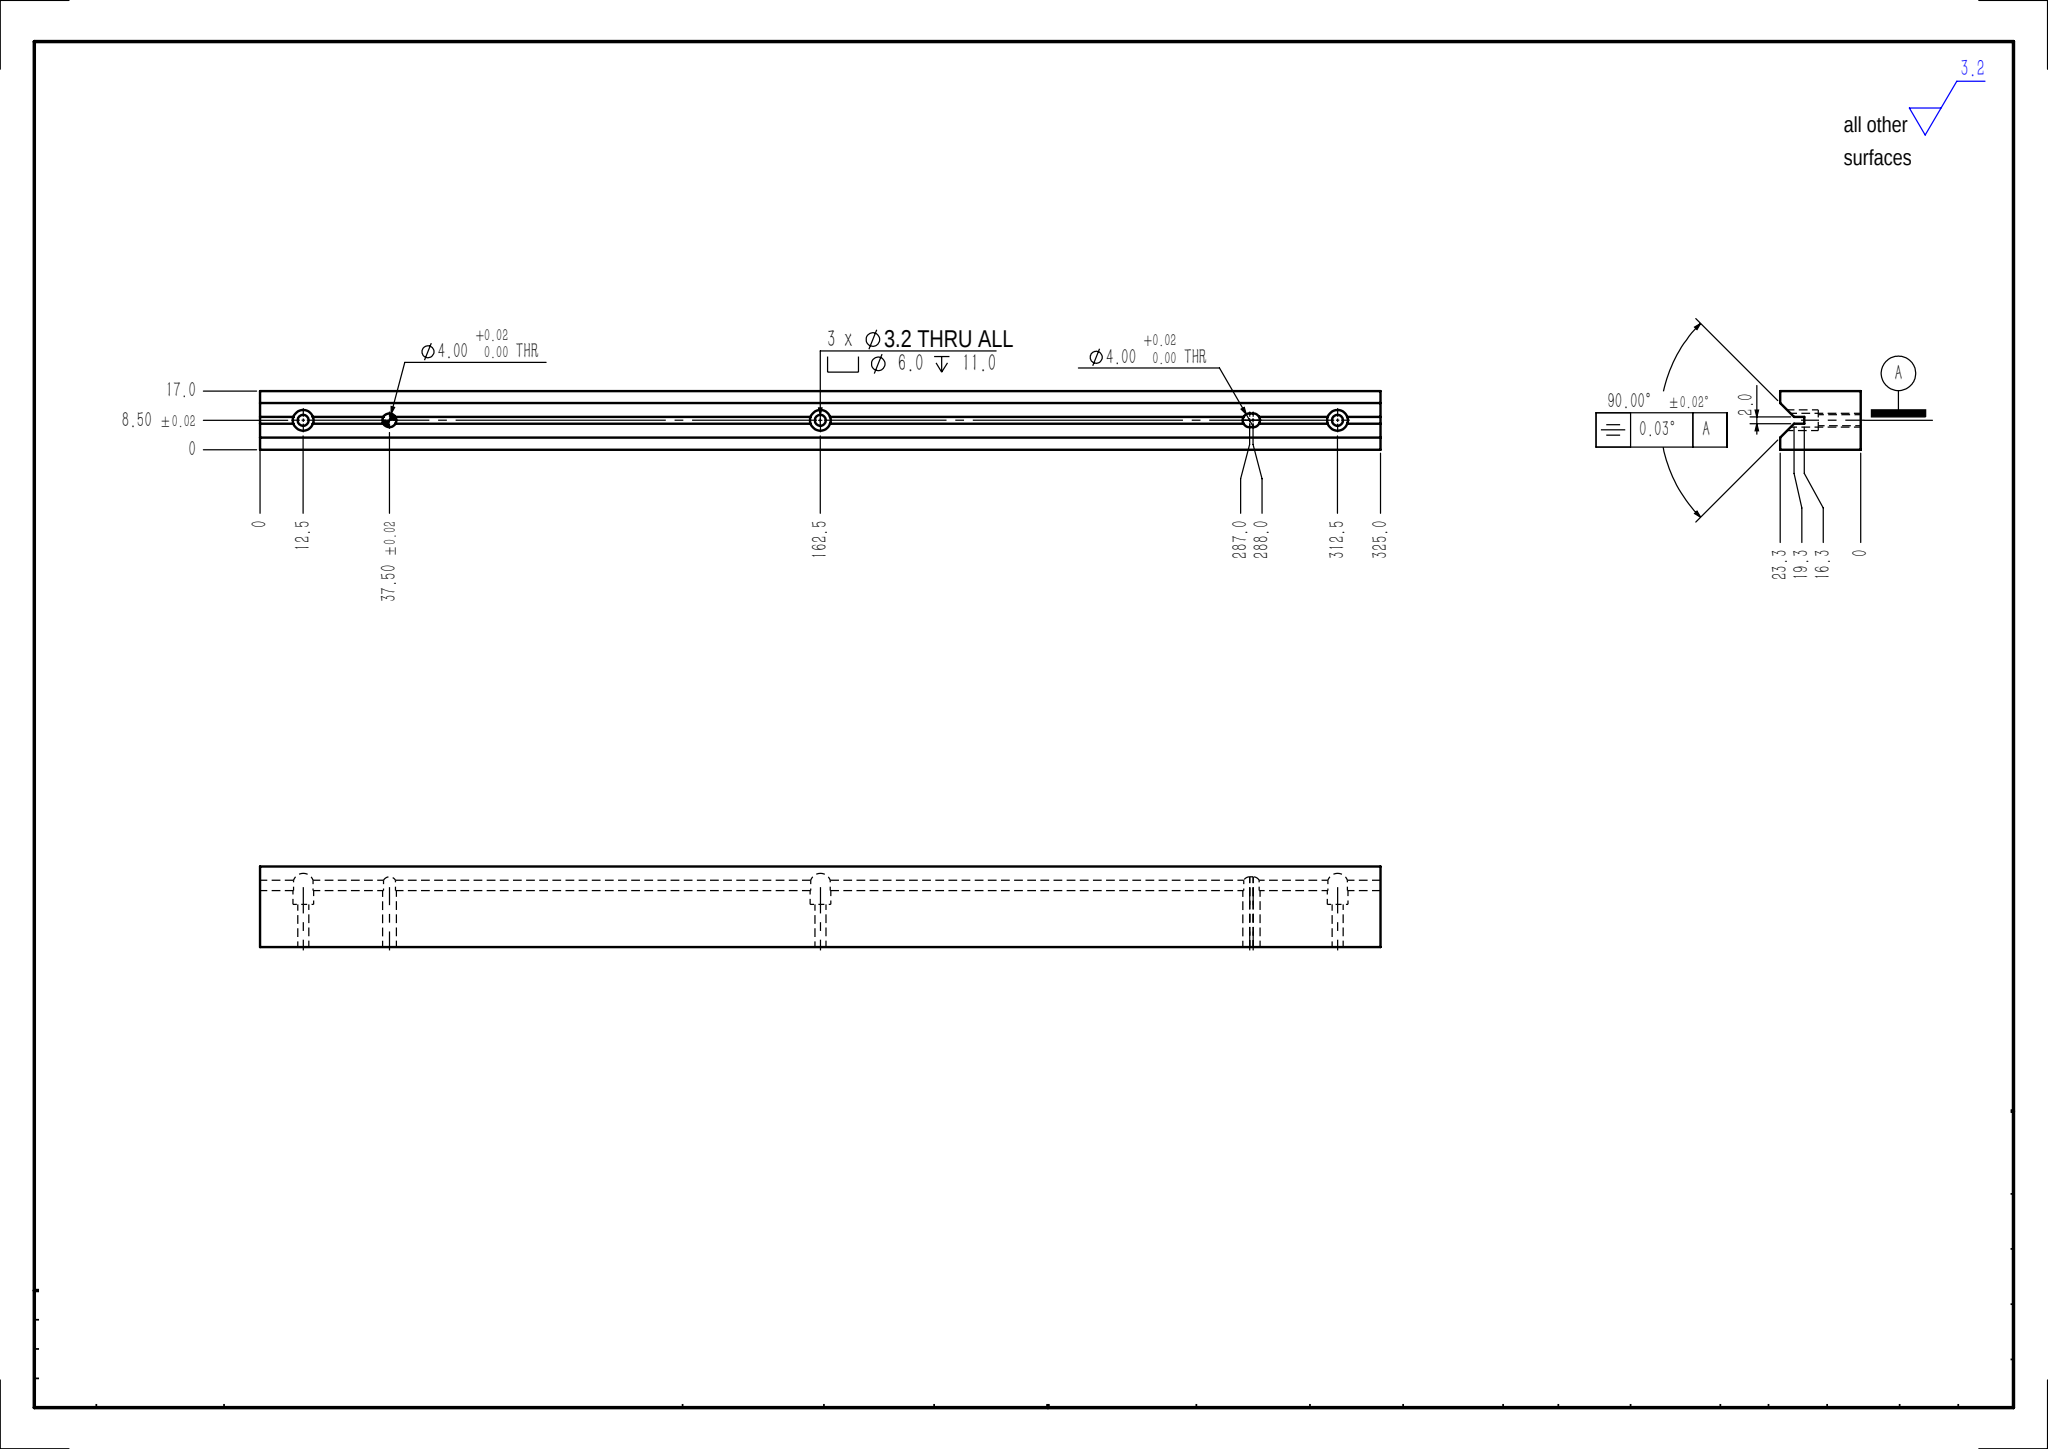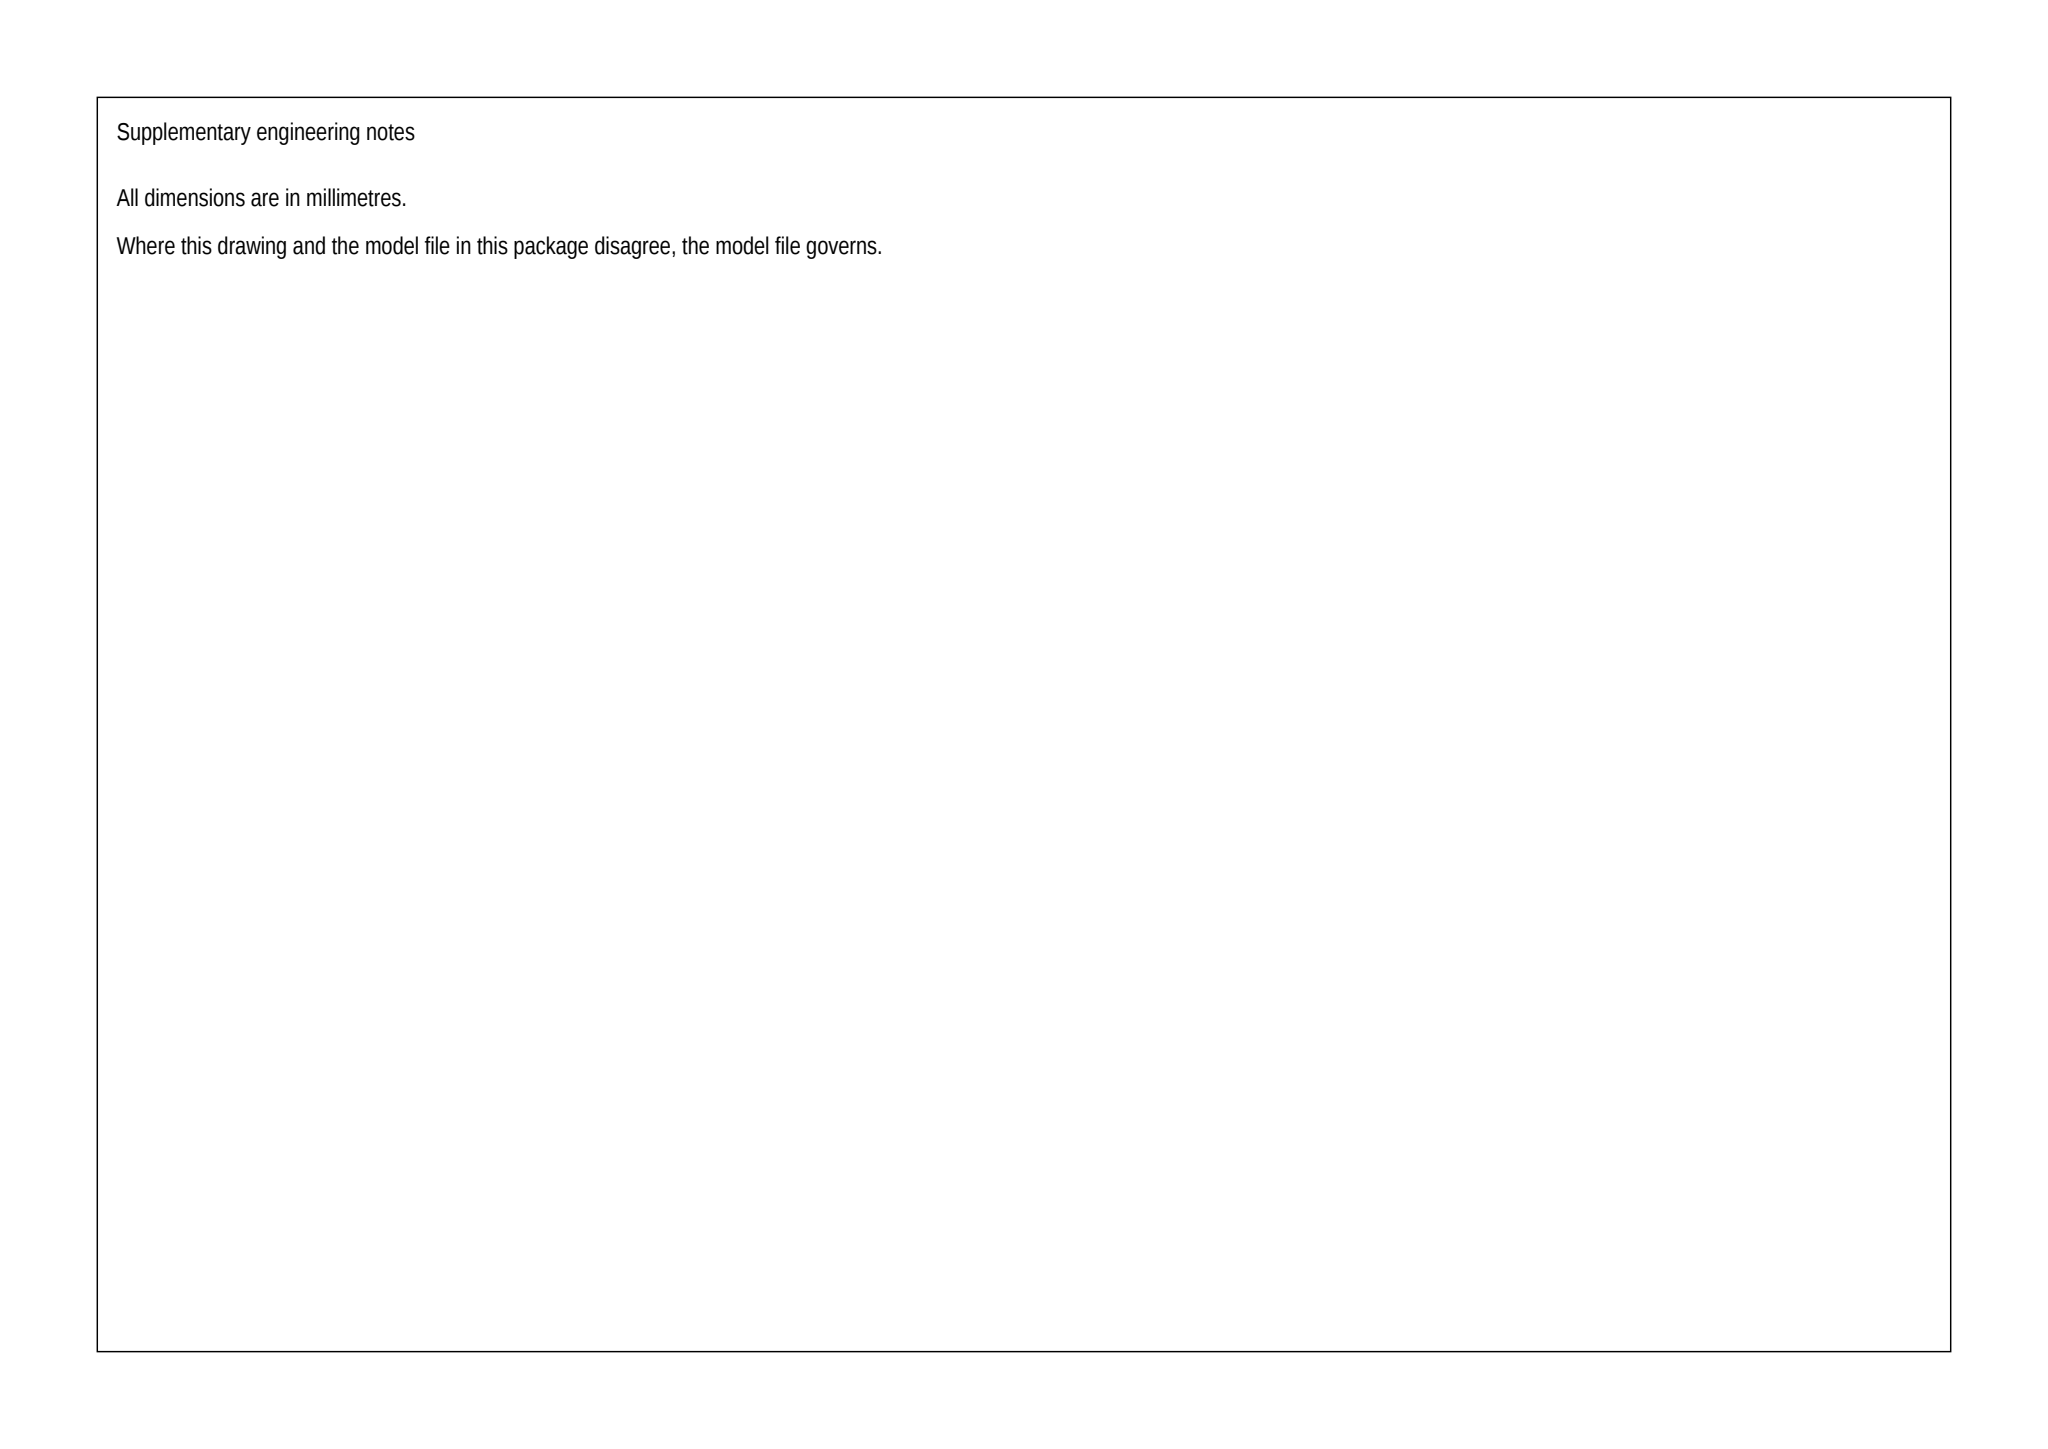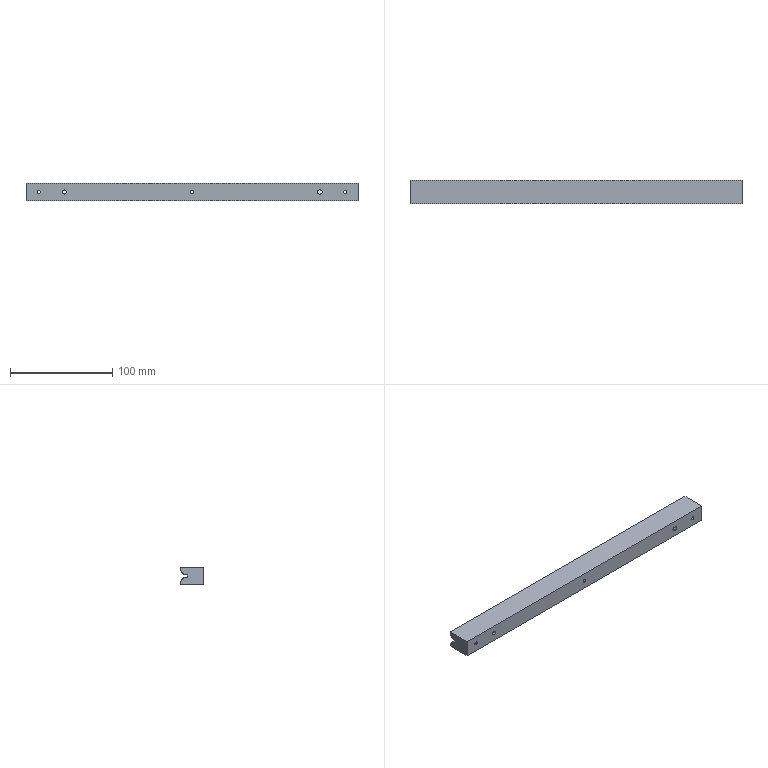Part | SolidWorks | mm | 1 solid | 48 faces | box 325 x 23.34 x 17 mm | volume 117860 mm3 | plane 32 | cylinder 16 | commonest cylinder face diameters 3.2 x6 6 x6 4 x4
build123d program:
from build123d import *

# Parameters (mm, degrees)
SKETCH1_W                                       = 325
SKETCH1_H                                       = 23.34
BOSS_EXTRUDE1_DEPTH                             = 8.5
CUT_EXTRUDE1_DEPTH                              = 326.321
M3_HEX_SOCKET_HEAD_CAP_SCREW_CBORE1_D           = 3.2
M3_HEX_SOCKET_HEAD_CAP_SCREW_CBORE1_CBORE_D     = 6
M3_HEX_SOCKET_HEAD_CAP_SCREW_CBORE1_CBORE_DEPTH = 11
SKETCH5_W                                       = 2
SKETCH5_H                                       = 3
CUT_EXTRUDE2_DEPTH                              = 326.321
LPATTERN1_COUNT                                 = 3
LPATTERN1_PITCH                                 = 150
SKETCH6_R                                       = 2
CUT_EXTRUDE3_DEPTH                              = 165.388


with BuildPart() as part:
    # Sketch1 → Boss-Extrude1 (new, symmetric)
    with BuildSketch(Plane.XY):
        Rectangle(SKETCH1_W, SKETCH1_H)
    extrude(amount=BOSS_EXTRUDE1_DEPTH, both=True)

    # Sketch2 → Cut-Extrude1 (cut, through all)
    with BuildSketch(Plane(origin=(162.5, 0, 0), x_dir=(0, 0, -1), z_dir=(1, 0, 0))):
        Polygon((-5, 11.67), (0, 6.67), (5, 11.67), align=None)
    extrude(amount=-CUT_EXTRUDE1_DEPTH, mode=Mode.SUBTRACT)

    # M3 Hex Socket Head Cap Screw CBORE1 (through all)
    with Locations(Plane(origin=(0, 11.67, 0), x_dir=(1, 0, 0), z_dir=(0, 1, 0))):
        with Locations((-150, 0)):
            m3_hex_socket_head_cap_screw_cbore1 = CounterBoreHole(M3_HEX_SOCKET_HEAD_CAP_SCREW_CBORE1_D / 2, M3_HEX_SOCKET_HEAD_CAP_SCREW_CBORE1_CBORE_D / 2, M3_HEX_SOCKET_HEAD_CAP_SCREW_CBORE1_CBORE_DEPTH)

    # Sketch5 → Cut-Extrude2 (cut, through all)
    with BuildSketch(Plane.ZY.offset(162.5)):
        with Locations((0, 6.17)):
            Rectangle(SKETCH5_W, SKETCH5_H)
    extrude(amount=-CUT_EXTRUDE2_DEPTH, mode=Mode.SUBTRACT)

    # LPattern1: M3 Hex Socket Head Cap Screw CBORE1 ×3
    with Locations(*[(i * LPATTERN1_PITCH, 0, 0) for i in range(1, LPATTERN1_COUNT)]):
        add(m3_hex_socket_head_cap_screw_cbore1, mode=Mode.SUBTRACT)

    # Sketch6 → Cut-Extrude3 (cut, through all)
    with BuildSketch(Plane(origin=(0, -11.67, 0), x_dir=(-1, 0, 0), z_dir=(0, -1, 0))):
        with Locations(Location((125, 0, 0), (0, 0, 90))):
            Circle(SKETCH6_R)
        with BuildLine():
            Line((-124.5, -2), (-125.5, -2))
            ThreePointArc((-125.5, -2), (-127.5, 0), (-125.5, 2))
            Line((-125.5, 2), (-124.5, 2))
            ThreePointArc((-124.5, 2), (-122.5, 0), (-124.5, -2))
        make_face()
    extrude(amount=-CUT_EXTRUDE3_DEPTH, mode=Mode.SUBTRACT)


solid = part.part